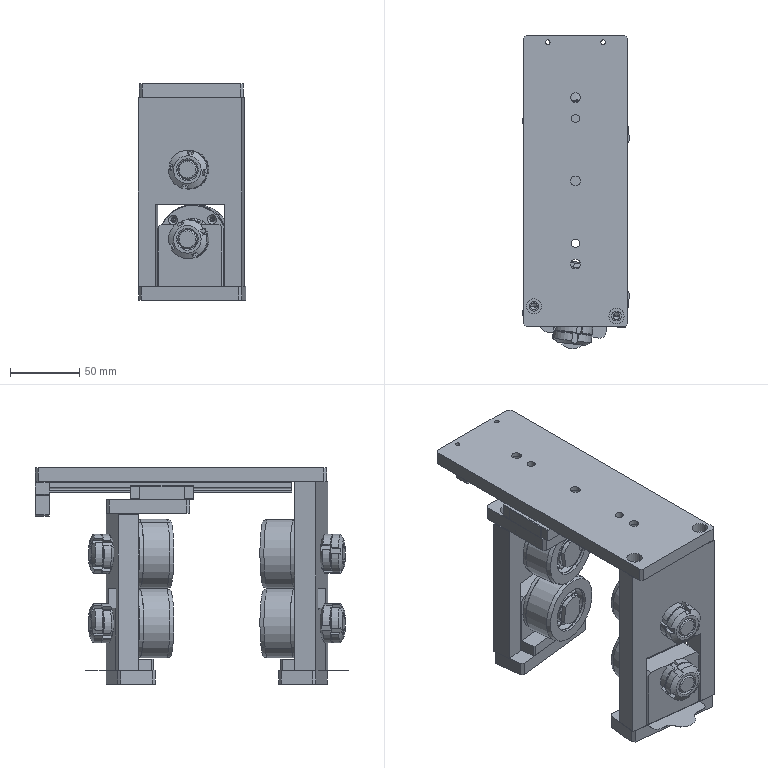Assembly | SolidWorks | mm | 47 component files | 47 solids | 2281 faces | box 77.4 x 225.88 x 156.2 mm | volume 745724 mm3 | plane 689 | cylinder 612 | torus 408 | cone 274 | sphere 224 | spline 74 | commonest cylinder face diameters 2.5 x72 6 x72 5 x36 17 x32 22.103 x32 3.4 x32 28 x32 3.5 x28
Bill of materials:
8TC-A17001-90-01PressureRollerSidePlate1 | 1 | #45 | Flat rectangular plate shaped like an upside-down U. It has a single round through-hole in the solid upper section, above an open rectangular slot that leaves two parallel legs. There are two small holes in the top end face.
8TC-A17001-90-02PressureRollerSidePlate2 | 1 | #45 | Flat plate shaped like an upside-down U, with a rectangular slot open at the bottom that forms two legs. It has a round through-hole in the solid upper section and two small holes in the top end face. The top corners appear to have small chamfers.
8TC-A17001-90-03PressureRollerMountingPlate2 | 1 | A3 | Thick rectangular plate with chamfered corners. It has two larger round through-holes near diagonally opposite corners and eight smaller round through-holes arranged in a 2 x 4 grid.
8TC-A17001-90-04PressureRollerMovingPlate | 2 | 45 | L-shaped block. A tall upright section has one large round through-hole, and a short, lower foot projects from one side at the base. The upper edges are chamfered.
8TC-A17001-90-05EdgePressingBasePlate | 1 | A3 | Long, thin rectangular plate with small chamfered corners. A row of round holes runs along the centerline, with two small holes at one end and two larger holes near the corners at the other end.
8TC-A17001-90-06EdgePressingRollerLockPlate | 2 | A3 | Rectangular block with chamfered corners and seven round through-holes of about three different sizes, arranged roughly symmetrically along its length.
8TC-A17001-90-07AdjustmentShim | 2 | SUS304 | Very thin flat plate, like a shim, with an irregular outline. One edge has two semicircular open slots and a rectangular notch between them, and the opposite side has a large rounded lobe. All corners are filleted.
8TC-A17001-90-08AdjustmentSeat | 1 | A3 | T-shaped block. A wide upper flange has two vertical round holes, and a narrower lower stem has two horizontal round through-holes of different diameters. The outer corners are chamfered.
8TC-A17001-91-01Spacer | 4 | A3 | Plain cylindrical ring or sleeve with a thin wall, a smooth outer surface and a smooth bore.
8TC-A17001-91-03Gland | 4 | A3 | Thin flat annular ring with a large central opening and four countersunk through-holes evenly spaced around the face.
8TC-A17001-91-04PressureRoller | 4 | Cr12MoV | Thick-walled cylindrical ring or sleeve. One end face has four small holes evenly spaced around it, there is an internal step or counterbore at the bore, and one outer end edge appears to be chamfered.
8TC-A17001-91-04PressureRollerAxis | 4 | 45 | Stepped cylindrical pin with a short, larger-diameter head at one end, a main shank and a smaller-diameter end section. The head appears to have a flat cut on one side.
GB292AngularContactBallBearing7003C | 8 | GCr15 | Annular assembly-like body with concentric outer and inner rings and a single row of spherical balls in the annular gap between them; looks like an open (unshielded) radial ball bearing.
GB812RoundNutM14_1.5 | 8 | A3 | Flat annular ring with a central round bore and six rectangular notches spaced around the outside edge; looks like a slotted ring or slotted round nut.
MGN12HGuideRail | 2 | 6061 Alloy | Long straight rail with a roughly rectangular cross-section, a row of evenly spaced counterbored-looking through-holes along the top, and grooves running along both sides; looks like a linear guide rail.
MGN12HSlider | 2 | 6061 Alloy | Rectangular block with a central U-shaped channel along its length, rounded bead or groove features on the channel side walls, and a stepped end-section; looks like a linear guide carriage or block body.
Mates:
1. coincident | 8TC-A17001-90-05EdgePressingBasePlate-1 plane at (0, 0, 0) dir (0, 0, 1) | assembly plane at (0, 0, 0) dir (0, 0, 1)
2. coincident | 8TC-A17001-90-05EdgePressingBasePlate-1 plane at (0, 0, 0) dir (0, 1, 0) | assembly plane at (0, 0, 0) dir (0, 1, 0)
3. coincident | 8TC-A17001-90-05EdgePressingBasePlate-1 plane at (0, 0, 0) dir (1, 0, 0) | assembly plane at (0, 0, 0) dir (1, 0, 0)
4. coincident | 8TC-A17001-90-05EdgePressingBasePlate-1 face at (0, 0, 0) dir (0, 0, -1) | 8TC-A17001-90-01PressureRollerSidePlate1-1 face at (37.914, -90.926, 0) dir (0, 0, 1)
5. concentric | 8TC-A17001-91-00UpperAndLowerPressAssembly-1/8TC-A17001-91-04PressureRollerAxis-1 face at (-2.947, -117.34, -52) dir (0.1167, 0.9932, 0) r 8.5 | 8TC-A17001-90-01PressureRollerSidePlate1-1 face at (0.6701, -86.551, -52) dir (0.1167, 0.9932, 0) r 8.5
6. coincident | 8TC-A17001-91-00UpperAndLowerPressAssembly-1/8TC-A17001-91-01Spacer-1 face at (0.6701, -86.551, -52) dir (-0.1167, -0.9932, 0) | 8TC-A17001-90-01PressureRollerSidePlate1-1 face at (0.6701, -86.551, -38.5) dir (0.1167, 0.9932, 0)
7. coincident | 8TC-A17001-91-00UpperAndLowerPressAssembly-1/8TC-A17001-91-04PressureRoller-1 face at (3.82, -59.736, -52) dir (0.1167, 0.9932, 0) | 8TC-A17001-91-00UpperAndLowerPressAssembly-2/8TC-A17001-91-04PressureRoller-1 face at (3.82, -59.736, -102.2) dir (0.1167, 0.9932, 0)
8. coincident | 8TC-A17001-90-05EdgePressingBasePlate-1 face at (0, 0, 0) dir (0, 0, -1) | MGN12H1R175Z0CGuideRailAssembly-1/MGN12HGuideRail-1 face at (-24, 7.5, 0) dir (0, 0, 1)
9. coincident | 8TC-A17001-90-03PressureRollerMountingPlate2-1 face at (0, 23.724, -13) dir (0, 0, 1) | MGN12H1R175Z0CGuideRailAssembly-1/MGN12HSlider-2 face at (-24, 13.724, -13) dir (0, 0, -1)
10. concentric | 8TC-A17001-90-03PressureRollerMountingPlate2-1 face at (-34, 3.724, -23) dir (0, 0, -1) r 3 | MGN12H1R175Z0CGuideRailAssembly-1/MGN12HSlider-2 face at (-34, 3.724, -13) dir (0, 0, -1) r 1.5
11. concentric | 8TC-A17001-90-03PressureRollerMountingPlate2-1 face at (-34, 23.724, -23) dir (0, 0, -1) r 3 | MGN12H1R175Z0CGuideRailAssembly-1/MGN12HSlider-2 face at (-34, 23.724, -13) dir (0, 0, -1) r 1.5
12. coincident | 8TC-A17001-90-02PressureRollerSidePlate2-1 face at (0.6701, 34.775, -50) dir (0.1167, -0.9932, 0) | 8TC-A17001-91-00UpperAndLowerPressAssembly-3/8TC-A17001-91-01Spacer-1 face at (0.6701, 34.775, -52) dir (-0.1167, 0.9932, 0)
13. concentric | 8TC-A17001-90-02PressureRollerSidePlate2-1 face at (-1.08, 49.673, -52) dir (-0.1167, 0.9932, 0) r 8.5 | 8TC-A17001-91-00UpperAndLowerPressAssembly-3/8TC-A17001-91-04PressureRollerAxis-1 face at (-2.947, 65.564, -52) dir (0.1167, -0.9932, 0) r 8.5
14. concentric | 8TC-A17001-91-00UpperAndLowerPressAssembly-2/8TC-A17001-91-04PressureRollerAxis-1 face at (-2.947, -117.34, -102.2) dir (0.1167, 0.9932, 0) r 8.5 | 8TC-A17001-90-04PressureRollerMovingPlate-1 face at (2.07, -74.633, -102.2) dir (-0.1167, -0.9932, 0) r 8.5
15. concentric | 8TC-A17001-91-00UpperAndLowerPressAssembly-4/8TC-A17001-91-04PressureRollerAxis-1 face at (-2.947, 65.564, -102.2) dir (0.1167, -0.9932, 0) r 8.5 | 8TC-A17001-90-04PressureRollerMovingPlate-2 face at (2.07, 22.857, -102.2) dir (-0.1167, 0.9932, 0) r 8.5
16. coincident | 8TC-A17001-91-00UpperAndLowerPressAssembly-3/8TC-A17001-91-04PressureRoller-1 face at (3.82, 7.96, -52) dir (0.1167, -0.9932, 0) | 8TC-A17001-91-00UpperAndLowerPressAssembly-4/8TC-A17001-91-04PressureRoller-1 face at (3.82, 7.96, -102.2) dir (0.1167, -0.9932, 0)
17. concentric | 8TC-A17001-90-03PressureRollerMountingPlate2-1 face at (14, 3.724, -23) dir (0, 0, -1) r 3 | MGN12H1R175Z0CGuideRailAssembly-2/MGN12HSlider-2 face at (14, 3.724, -13) dir (0, 0, -1) r 1.5
18. concentric | 8TC-A17001-90-03PressureRollerMountingPlate2-1 face at (34, 3.724, -23) dir (0, 0, -1) r 3 | MGN12H1R175Z0CGuideRailAssembly-2/MGN12HSlider-2 face at (34, 3.724, -13) dir (0, 0, -1) r 1.5
19. coincident | 8TC-A17001-90-03PressureRollerMountingPlate2-1 face at (0, 23.724, -13) dir (0, 0, 1) | MGN12H1R175Z0CGuideRailAssembly-2/MGN12HSlider-2 face at (24, 13.724, -13) dir (0, 0, -1)
20. coincident | 8TC-A17001-90-05EdgePressingBasePlate-1 face at (0, 0, 0) dir (0, 0, -1) | 8TC-A17001-90-08AdjustmentSeat-1 face at (25, 105, 0) dir (0, 0, 1)
21. coincident | 8TC-A17001-90-05EdgePressingBasePlate-1 face at (37.5, 105, 10) dir (0, 1, 0) | 8TC-A17001-90-08AdjustmentSeat-1 face at (0, 105, 0) dir (0, 1, 0)
22. width | 8TC-A17001-90-08AdjustmentSeat-1 face at (-25, 105, -10) dir (-1, 0, 0) | 8TC-A17001-90-08AdjustmentSeat-1 face at (25, 105, -10) dir (1, 0, 0) | 8TC-A17001-90-05EdgePressingBasePlate-1 face at (37.5, 105, 10) dir (1, 0, 0) | 8TC-A17001-90-05EdgePressingBasePlate-1 face at (-37.5, 105, 10) dir (-1, 0, 0)
23. coincident | MGN12H1R175Z0CGuideRailAssembly-1/MGN12HGuideRail-1 face at (-18, 95, -8) dir (0, 1, 0) | MGN12H1R175Z0CGuideRailAssembly-2/MGN12HGuideRail-1 face at (30, 95, -8) dir (0, 1, 0)
24. concentric | 8TC-A17001-90-05EdgePressingBasePlate-1 face at (-30, -90.5, 10) dir (0, 0, 1) r 3.5 | 8TC-A17001-90-01PressureRollerSidePlate1-1 face at (-30, -90.5, 0) dir (0, 0, 1) r 2.5
25. distance | 8TC-A17001-91-00UpperAndLowerPressAssembly-1/8TC-A17001-91-04PressureRoller-1 face at (3.82, -59.736, -52) dir (-0.1167, -0.9932, 0) r 25 | 8TC-A17001-91-00UpperAndLowerPressAssembly-2/8TC-A17001-91-04PressureRoller-1 face at (3.82, -59.736, -102.2) dir (-0.1167, -0.9932, 0) r 25
26. coincident | 8TC-A17001-90-02PressureRollerSidePlate2-1 face at (-0.2049, 42.224, -136.2) dir (0, 0, -1) | 8TC-A17001-90-06EdgePressingRollerLockPlate-2 face at (0.4951, 36.265, -136.2) dir (0, 0, 1)
27. concentric | 8TC-A17001-90-02PressureRollerSidePlate2-1 face at (-30, 38.724, -136.2) dir (0, 0, -1) r 2.5 | 8TC-A17001-90-06EdgePressingRollerLockPlate-2 face at (-30, 38.724, -146.2) dir (0, 0, -1) r 3.3
28. concentric | 8TC-A17001-90-02PressureRollerSidePlate2-1 face at (29.59, 45.724, -136.2) dir (0, 0, -1) r 2.5 | 8TC-A17001-90-06EdgePressingRollerLockPlate-2 face at (29.59, 45.724, -146.2) dir (0, 0, -1) r 3.3
29. concentric | 8TC-A17001-90-05EdgePressingBasePlate-1 face at (-24, 85, 0) dir (0, 0, -1) r 1.25 | MGN12H1R175Z0CGuideRailAssembly-1/MGN12HGuideRail-1 face at (-24, 85, -8) dir (0, 0, -1) r 3
30. concentric | 8TC-A17001-90-05EdgePressingBasePlate-1 face at (24, 85, 0) dir (0, 0, -1) r 1.25 | MGN12H1R175Z0CGuideRailAssembly-2/MGN12HGuideRail-1 face at (24, 85, -8) dir (0, 0, -1) r 3
31. concentric | 8TC-A17001-90-02PressureRollerSidePlate2-1 face at (-30, 38.724, -23) dir (0, 0, 1) r 2.5 | 8TC-A17001-90-03PressureRollerMountingPlate2-1 face at (-30, 38.724, -13) dir (0, 0, 1) r 3.5
32. concentric | 8TC-A17001-90-03PressureRollerMountingPlate2-1 face at (29.59, 45.724, -13) dir (0, 0, 1) r 3.5 | 8TC-A17001-90-02PressureRollerSidePlate2-1 face at (29.59, 45.724, -23) dir (0, 0, 1) r 2.5
33. coincident | 8TC-A17001-90-03PressureRollerMountingPlate2-1 face at (0, 23.724, -23) dir (0, 0, -1) | 8TC-A17001-90-02PressureRollerSidePlate2-1 face at (36.164, 54.048, -23) dir (0, 0, 1)
34. concentric | 8TC-A17001-90-05EdgePressingBasePlate-1 face at (29.59, -97.5, 10) dir (0, 0, 1) r 5.5 | 8TC-A17001-90-01PressureRollerSidePlate1-1 face at (29.59, -97.5, 0) dir (0, 0, 1) r 2.5
35. coincident | 8TC-A17001-90-04PressureRollerMovingPlate-2 face at (22.756, 52.473, -136.2) dir (0, 0, -1) | 8TC-A17001-90-06EdgePressingRollerLockPlate-2 face at (0.4951, 36.265, -136.2) dir (0, 0, 1)
36. concentric | 8TC-A17001-90-06EdgePressingRollerLockPlate-2 face at (18.517, 32.844, -146.2) dir (0, 0, -1) r 3 | 8TC-A17001-90-04PressureRollerMovingPlate-2 face at (18.517, 32.844, -136.2) dir (0, 0, -1) r 3
37. concentric | 8TC-A17001-90-06EdgePressingRollerLockPlate-2 face at (-16.244, 28.761, -146.2) dir (0, 0, -1) r 3 | 8TC-A17001-90-04PressureRollerMovingPlate-2 face at (-16.244, 28.761, -136.2) dir (0, 0, -1) r 3
38. coincident | 8TC-A17001-90-06EdgePressingRollerLockPlate-2 face at (0.4951, 36.265, -136.2) dir (0, 0, 1) | 8TC-A17001-90-07AdjustmentShim-2 face at (-17.585, 40.183, -136.2) dir (0, 0, -1)
39. coincident | 8TC-A17001-90-07AdjustmentShim-1 face at (17.176, -96.042, -136.2) dir (0, 0, -1) | 8TC-A17001-90-07AdjustmentShim-2 face at (-17.585, 40.183, -136.2) dir (0, 0, -1)
40. coincident | 8TC-A17001-90-01PressureRollerSidePlate1-1 face at (-0.2049, -94, -136.2) dir (0, 0, -1) | 8TC-A17001-90-06EdgePressingRollerLockPlate-1 face at (0.4951, -88.041, -136.2) dir (0, 0, 1)
41. concentric | 8TC-A17001-90-01PressureRollerSidePlate1-1 face at (-30, -90.5, -136.2) dir (0, 0, -1) r 2.5 | 8TC-A17001-90-06EdgePressingRollerLockPlate-1 face at (-30, -90.5, -146.2) dir (0, 0, -1) r 3.3
42. concentric | 8TC-A17001-90-01PressureRollerSidePlate1-1 face at (29.59, -97.5, -136.2) dir (0, 0, -1) r 2.5 | 8TC-A17001-90-06EdgePressingRollerLockPlate-1 face at (29.59, -97.5, -146.2) dir (0, 0, -1) r 3.3
43. concentric | 8TC-A17001-90-04PressureRollerMovingPlate-1 face at (17.176, -96.042, -136.2) dir (0, 0, -1) r 2.5 | 8TC-A17001-90-06EdgePressingRollerLockPlate-1 face at (17.176, -96.042, -146.2) dir (0, 0, -1) r 3.3
44. concentric | 8TC-A17001-91-04PressureRollerAxis-1 face at (-71.146, -78.224, 33.126) dir (0.03452, 0.999, 0.02904) r 8.5 | 8TC-A17001-91-01Spacer-1 face at (-69.903, -42.261, 34.171) dir (-0.03452, -0.999, -0.02904) r 10.5
45. concentric | 8TC-A17001-91-04PressureRoller-1 face at (-69.144, -20.283, 34.81) dir (-0.03452, -0.999, -0.02904) r 25 | 8TC-A17001-91-03Gland-1 face at (-69.903, -42.261, 34.171) dir (-0.03452, -0.999, -0.02904) r 24.5
46. concentric | 8TC-A17001-91-04PressureRoller-1 face at (-50.801, -43.091, 40.038) dir (-0.03452, -0.999, -0.02904) r 1.25 | 8TC-A17001-91-03Gland-1 face at (-50.904, -46.088, 39.95) dir (-0.03452, -0.999, -0.02904) r 1.7
47. coincident | GB812RoundNutM14_1.5-1 face at (-70.869, -70.232, 33.358) dir (-0.03452, -0.999, -0.02904) | GB812RoundNutM14_1.5-2 face at (-70.869, -70.232, 33.358) dir (0.03452, 0.999, 0.02904)
48. concentric | 8TC-A17001-91-04PressureRollerAxis-1 face at (-69.109, -19.284, 34.839) dir (0.03452, 0.999, 0.02904) r 7 | GB812RoundNutM14_1.5-1 face at (-70.869, -70.232, 33.358) dir (0.03452, 0.999, 0.02904) r 7
49. concentric | 8TC-A17001-91-04PressureRollerAxis-1 face at (-69.109, -19.284, 34.839) dir (0.03452, 0.999, 0.02904) r 7 | GB812RoundNutM14_1.5-2 face at (-70.869, -70.232, 33.358) dir (-0.03452, -0.999, -0.02904) r 7
50. distance | GB812RoundNutM14_1.5-1 face at (-70.593, -62.24, 33.59) dir (0.03452, 0.999, 0.02904) | 8TC-A17001-91-04PressureRollerAxis-1 face at (-76.414, -60.928, 29.795) dir (-0.03452, -0.999, -0.02904)
51. concentric | 8TC-A17001-91-04PressureRoller-1 face at (-69.144, -20.283, 34.81) dir (-0.03452, -0.999, -0.02904) r 17.5 | 8TC-A17001-91-04PressureRollerAxis-1 face at (-71.146, -78.224, 33.126) dir (0.03452, 0.999, 0.02904) r 8.5
52. coincident | 8TC-A17001-91-04PressureRoller-1 face at (-69.903, -42.261, 34.171) dir (-0.03452, -0.999, -0.02904) | 8TC-A17001-91-03Gland-1 face at (-69.903, -42.261, 34.171) dir (0.03452, 0.999, 0.02904)
53. concentric | 8TC-A17001-91-04PressureRollerAxis-1 face at (-71.146, -78.224, 33.126) dir (0.03452, 0.999, 0.02904) r 8.5 | 8TC-A17001-91-01Spacer-1 face at (-69.903, -42.261, 34.171) dir (-0.03452, -0.999, -0.02904) r 10.5
54. coincident | GB292AngularContactBallBearing7003C-1 face at (-72.094, -32.686, 51.772) dir (0.03452, 0.999, 0.02904) | GB292AngularContactBallBearing7003C-2 face at (-84.136, -32.049, 44.141) dir (-0.03452, -0.999, -0.02904)
55. concentric | GB292AngularContactBallBearing7003C-1 face at (-69.558, -32.271, 34.461) dir (0.03452, 0.999, 0.02904) r 17.5 | GB292AngularContactBallBearing7003C-2 face at (-69.558, -32.271, 34.461) dir (-0.03452, -0.999, -0.02904) r 17.5
56. concentric | 8TC-A17001-91-04PressureRoller-1 face at (-69.144, -20.283, 34.81) dir (-0.03452, -0.999, -0.02904) r 17.5 | GB292AngularContactBallBearing7003C-2 face at (-69.558, -32.271, 34.461) dir (-0.03452, -0.999, -0.02904) r 17.5
57. coincident | 8TC-A17001-91-04PressureRoller-1 face at (-69.213, -22.281, 34.752) dir (-0.03452, -0.999, -0.02904) | GB292AngularContactBallBearing7003C-2 face at (-83.79, -22.059, 44.431) dir (0.03452, 0.999, 0.02904)
58. coincident | 8TC-A17001-91-04PressureRollerAxis-1 face at (-69.213, -22.281, 34.752) dir (-0.03452, -0.999, -0.02904) | GB292AngularContactBallBearing7003C-2 face at (-76.293, -22.173, 39.453) dir (0.03452, 0.999, 0.02904)
59. coincident | GB292AngularContactBallBearing7003C-1 face at (-71.135, -42.463, 42.579) dir (-0.03452, -0.999, -0.02904) | 8TC-A17001-91-01Spacer-1 face at (-69.903, -42.261, 34.171) dir (0.03452, 0.999, 0.02904)
60. concentric | MGN12HSlider-2 face at (-6, 5.5, -15.45) dir (0, 0, 1) r 1.25 | MGN12HGuideRail-1 face at (-6, 5.5, -87.5) dir (0, 0, -1) r 1.25
61. concentric | MGN12HSlider-2 face at (6, 5.5, -15.45) dir (0, 0, 1) r 1.25 | MGN12HGuideRail-1 face at (6, 5.5, -87.5) dir (0, 0, -1) r 1.25